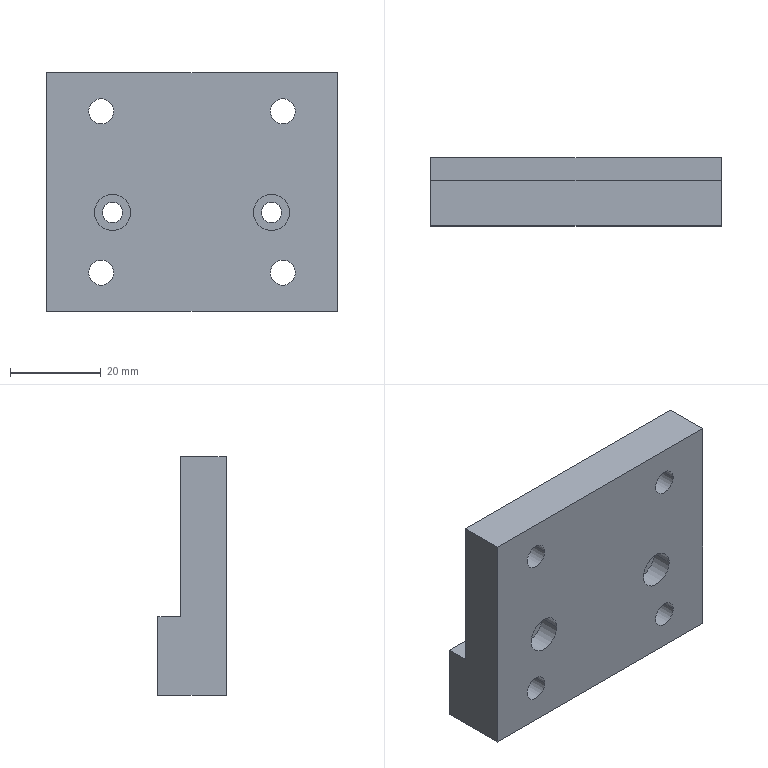Component | SolidWorks | RotaryCylinderSupport-1 | 1 solid | 38 faces | box 64 x 15 x 52.5 mm | volume 36049 mm3 | cylinder 24 | plane 14 | commonest cylinder face diameters 10 x8 5.5 x8 8 x4 4.5 x4
build123d program:
from build123d import *

# Parameters (mm, degrees)
SKETCH2_W                                       = 64
SKETCH2_H                                       = 52.5
BOSS_EXTRUDE1_DEPTH                             = 10
M4_HEX_SOCKET_HEAD_CAP_SCREW_CBORE1_D           = 4.5
M4_HEX_SOCKET_HEAD_CAP_SCREW_CBORE1_DEPTH       = 20
M4_HEX_SOCKET_HEAD_CAP_SCREW_CBORE1_CBORE_D     = 8
M4_HEX_SOCKET_HEAD_CAP_SCREW_CBORE1_CBORE_DEPTH = 4.6
M4_HEX_SOCKET_HEAD_CAP_SCREW_CBORE1_TIP         = 1.352
SKETCH5_W                                       = 64
SKETCH5_H                                       = 17.25
BOSS_EXTRUDE2_DEPTH                             = 5
M5_HEX_SOCKET_HEAD_CAP_SCREW_CBORE2_D           = 5.5
M5_HEX_SOCKET_HEAD_CAP_SCREW_CBORE2_DEPTH       = 20
M5_HEX_SOCKET_HEAD_CAP_SCREW_CBORE2_CBORE_D     = 10
M5_HEX_SOCKET_HEAD_CAP_SCREW_CBORE2_CBORE_DEPTH = 5.7
M5_HEX_SOCKET_HEAD_CAP_SCREW_CBORE2_TIP         = 1.652
M5_HEX_SOCKET_HEAD_CAP_SCREW_CBORE3_D           = 5.5
M5_HEX_SOCKET_HEAD_CAP_SCREW_CBORE3_DEPTH       = 20
M5_HEX_SOCKET_HEAD_CAP_SCREW_CBORE3_CBORE_D     = 10
M5_HEX_SOCKET_HEAD_CAP_SCREW_CBORE3_CBORE_DEPTH = 5.7
M5_HEX_SOCKET_HEAD_CAP_SCREW_CBORE3_TIP         = 1.652


with BuildPart() as part:
    # Sketch2 → Boss-Extrude1 (new body)
    with BuildSketch(Plane.XY):
        with Locations((0, 9)):
            Rectangle(SKETCH2_W, SKETCH2_H)
    extrude(amount=BOSS_EXTRUDE1_DEPTH)

    # M4 Hex Socket Head Cap Screw CBORE1
    with Locations(Plane.XY.offset(10)):
        with Locations((-17.5, 4.5), (17.5, 4.5)):
            CounterBoreHole(M4_HEX_SOCKET_HEAD_CAP_SCREW_CBORE1_D / 2, M4_HEX_SOCKET_HEAD_CAP_SCREW_CBORE1_CBORE_D / 2, M4_HEX_SOCKET_HEAD_CAP_SCREW_CBORE1_CBORE_DEPTH, depth=M4_HEX_SOCKET_HEAD_CAP_SCREW_CBORE1_DEPTH)
            with Locations((0, 0, -(M4_HEX_SOCKET_HEAD_CAP_SCREW_CBORE1_DEPTH + M4_HEX_SOCKET_HEAD_CAP_SCREW_CBORE1_TIP / 2))):  # 118° drill point
                Cone(0, M4_HEX_SOCKET_HEAD_CAP_SCREW_CBORE1_D / 2, M4_HEX_SOCKET_HEAD_CAP_SCREW_CBORE1_TIP, mode=Mode.SUBTRACT)

    # Sketch5 → Boss-Extrude2 (add)
    with BuildSketch(Plane(origin=(0, 0, 0), x_dir=(-1, 0, 0), z_dir=(0, 0, -1))):
        with Locations((0, -8.625)):
            Rectangle(SKETCH5_W, SKETCH5_H)
    extrude(amount=BOSS_EXTRUDE2_DEPTH)

    # M5 Hex Socket Head Cap Screw CBORE2
    with Locations(Plane(origin=(0, 0, -5), x_dir=(-1, 0, 0), z_dir=(0, 0, -1))):
        with Locations((-20, -8.75), (20, -8.75)):
            CounterBoreHole(M5_HEX_SOCKET_HEAD_CAP_SCREW_CBORE2_D / 2, M5_HEX_SOCKET_HEAD_CAP_SCREW_CBORE2_CBORE_D / 2, M5_HEX_SOCKET_HEAD_CAP_SCREW_CBORE2_CBORE_DEPTH, depth=M5_HEX_SOCKET_HEAD_CAP_SCREW_CBORE2_DEPTH)
            with Locations((0, 0, -(M5_HEX_SOCKET_HEAD_CAP_SCREW_CBORE2_DEPTH + M5_HEX_SOCKET_HEAD_CAP_SCREW_CBORE2_TIP / 2))):  # 118° drill point
                Cone(0, M5_HEX_SOCKET_HEAD_CAP_SCREW_CBORE2_D / 2, M5_HEX_SOCKET_HEAD_CAP_SCREW_CBORE2_TIP, mode=Mode.SUBTRACT)

    # M5 Hex Socket Head Cap Screw CBORE3
    with Locations(Plane(origin=(0, 0, 0), x_dir=(-1, 0, 0), z_dir=(0, 0, -1))):
        with Locations((-20, 26.75), (20, 26.75)):
            CounterBoreHole(M5_HEX_SOCKET_HEAD_CAP_SCREW_CBORE3_D / 2, M5_HEX_SOCKET_HEAD_CAP_SCREW_CBORE3_CBORE_D / 2, M5_HEX_SOCKET_HEAD_CAP_SCREW_CBORE3_CBORE_DEPTH, depth=M5_HEX_SOCKET_HEAD_CAP_SCREW_CBORE3_DEPTH)
            with Locations((0, 0, -(M5_HEX_SOCKET_HEAD_CAP_SCREW_CBORE3_DEPTH + M5_HEX_SOCKET_HEAD_CAP_SCREW_CBORE3_TIP / 2))):  # 118° drill point
                Cone(0, M5_HEX_SOCKET_HEAD_CAP_SCREW_CBORE3_D / 2, M5_HEX_SOCKET_HEAD_CAP_SCREW_CBORE3_TIP, mode=Mode.SUBTRACT)


solid = part.part

# Placed as in the assembly
solid = solid.moved(Location((-331.696, -98.151, 336.468), (90, 0, 0)))